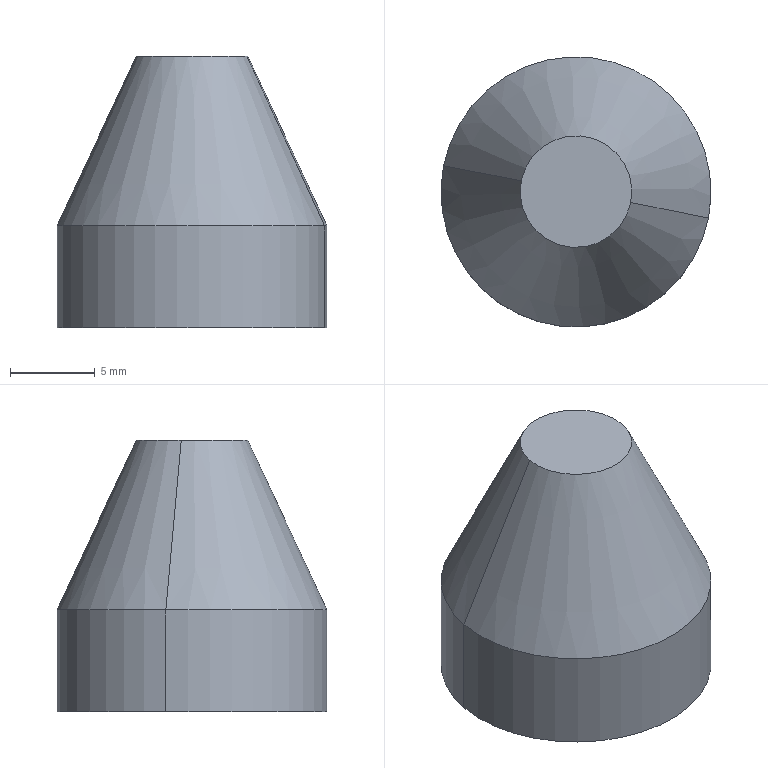Component | SolidWorks | DC-46-016-1 | 1 solid | 10 faces | box 15.9 x 15.9 x 16 mm | volume 2053 mm3 | cone 4 | cylinder 4 | plane 2 | commonest cylinder face diameters 5 x2 15.9 x2
build123d program:
from build123d import *

# Parameters (mm, degrees)
SKETCH1_R             = 7.95
BOSS_EXTRUDE1_DEPTH   = 8
M6_TAPPED_HOLE1_D     = 5
M6_TAPPED_HOLE1_DEPTH = 9
M6_TAPPED_HOLE1_TIP   = 1.502
CHAMFER1_SIZE         = 10
CHAMFER1_SIZE2        = 4.663


with BuildPart() as part:
    # Sketch1 → Boss-Extrude1 (new, symmetric)
    with BuildSketch(Plane.XY):
        Circle(SKETCH1_R)
    extrude(amount=BOSS_EXTRUDE1_DEPTH, both=True)

    # M6 Tapped Hole1
    with Locations(Plane(origin=(0, 0, -8), x_dir=(-1, 0, 0), z_dir=(0, 0, -1))):
        with Locations((0, 0)):
            Hole(M6_TAPPED_HOLE1_D / 2, depth=M6_TAPPED_HOLE1_DEPTH)
            with Locations((0, 0, -(M6_TAPPED_HOLE1_DEPTH + M6_TAPPED_HOLE1_TIP / 2))):  # 118° drill point
                Cone(0, M6_TAPPED_HOLE1_D / 2, M6_TAPPED_HOLE1_TIP, mode=Mode.SUBTRACT)

    # Chamfer1
    chamfer1_edges = [part.edges().sort_by_distance(p)[0] for p in [
        (-7.95, 0, 8),
    ]]
    chamfer1_side = [part.faces().sort_by_distance(p)[0] for p in [
        (-7.95, 0, 0),
    ]]
    chamfer(chamfer1_edges, length=CHAMFER1_SIZE, length2=CHAMFER1_SIZE2, reference=chamfer1_side[0])


solid = part.part

# Placed as in the assembly
solid = solid.moved(Location((271.865, 115.227, 2096.633), (0, 0, 0)))